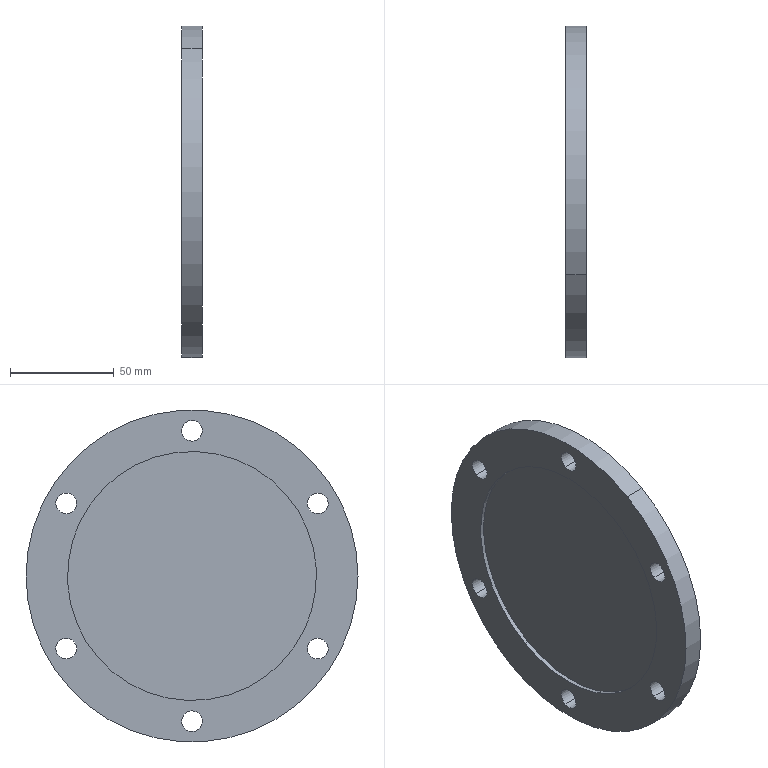Component | SolidWorks | GearboxEndCover-NoHole-2 | 1 solid | 19 faces | box 10 x 160 x 160 mm | volume 173730 mm3 | cylinder 16 | plane 3 | commonest cylinder face diameters 10 x12 120 x2 160 x2
build123d program:
from build123d import *

# Parameters (mm, degrees)
SKETCH1_3_R         = 80
SKETCH1_3_R_2       = 5
BOSS_EXTRUDE1_DEPTH = 8
BOSS_EXTRUDE2_START = -2
SKETCH1_3_2_R       = 80
SKETCH1_3_2_R_2     = 60
SKETCH1_3_2_R_3     = 5
BOSS_EXTRUDE2_DEPTH = 2


with BuildPart() as part:
    # Sketch1_3 → Boss-Extrude1 (new body)
    with BuildSketch(Plane(origin=(0, 0, 0), x_dir=(1, 0, 0), z_dir=(0, 1, 0))):
        with Locations(Location((0, 0, 0), (0, 0, 270))):
            Circle(SKETCH1_3_R)
        with Locations(Location((70, 0, 0), (0, 0, 270))):
            Circle(SKETCH1_3_R_2, mode=Mode.SUBTRACT)
        with Locations(Location((35, -60.622, 0), (0, 0, 270))):
            Circle(SKETCH1_3_R_2, mode=Mode.SUBTRACT)
        with Locations(Location((-35, -60.622, 0), (0, 0, 270))):
            Circle(SKETCH1_3_R_2, mode=Mode.SUBTRACT)
        with Locations(Location((-70, 0, 0), (0, 0, 270))):
            Circle(SKETCH1_3_R_2, mode=Mode.SUBTRACT)
        with Locations(Location((-35, 60.622, 0), (0, 0, 270))):
            Circle(SKETCH1_3_R_2, mode=Mode.SUBTRACT)
        with Locations(Location((35, 60.622, 0), (0, 0, 270))):
            Circle(SKETCH1_3_R_2, mode=Mode.SUBTRACT)
    extrude(amount=BOSS_EXTRUDE1_DEPTH)

    # Sketch1_3 2 → Boss-Extrude2 (add)
    with BuildSketch(Plane(origin=(0, 0, 0), x_dir=(1, 0, 0), z_dir=(0, 1, 0)).offset(BOSS_EXTRUDE2_START)):
        with Locations(Location((0, 0, 0), (0, 0, 270))):
            Circle(SKETCH1_3_2_R)
        with Locations(Location((0, 0, 0), (0, 0, 270))):
            Circle(SKETCH1_3_2_R_2, mode=Mode.SUBTRACT)
        with Locations(Location((70, 0, 0), (0, 0, 270))):
            Circle(SKETCH1_3_2_R_3, mode=Mode.SUBTRACT)
        with Locations(Location((35, -60.622, 0), (0, 0, 270))):
            Circle(SKETCH1_3_2_R_3, mode=Mode.SUBTRACT)
        with Locations(Location((-35, -60.622, 0), (0, 0, 270))):
            Circle(SKETCH1_3_2_R_3, mode=Mode.SUBTRACT)
        with Locations(Location((-70, 0, 0), (0, 0, 270))):
            Circle(SKETCH1_3_2_R_3, mode=Mode.SUBTRACT)
        with Locations(Location((-35, 60.622, 0), (0, 0, 270))):
            Circle(SKETCH1_3_2_R_3, mode=Mode.SUBTRACT)
        with Locations(Location((35, 60.622, 0), (0, 0, 270))):
            Circle(SKETCH1_3_2_R_3, mode=Mode.SUBTRACT)
    extrude(amount=BOSS_EXTRUDE2_DEPTH)


solid = part.part

# Placed as in the assembly
solid = solid.moved(Location((-178.429, -8.561, -165), (90, 0, -90)))
STEP:
#1=CARTESIAN_POINT('',(-7.104,0.844,-8.542));
#2=VERTEX_POINT('',#1);
#3=CARTESIAN_POINT('',(-7.104,-1.518,-4.45));
#4=VERTEX_POINT('',#3);
#5=CARTESIAN_POINT('',(-7.104,-0.3371,-6.496));
#6=DIRECTION('',(1.,0.,-0.));
#7=DIRECTION('',(0.,-0.5,0.866));
#8=AXIS2_PLACEMENT_3D('',#5,#6,#7);
#9=CIRCLE('',#8,2.362);
#10=EDGE_CURVE('',#2,#4,#9,.T.);
#11=ORIENTED_EDGE('',*,*,#10,.F.);
#12=CARTESIAN_POINT('',(-7.025,0.844,-8.542));
#13=VERTEX_POINT('',#12);
#14=CARTESIAN_POINT('',(-7.104,0.844,-8.542));
#15=DIRECTION('',(1.,0.,-0.));
#16=VECTOR('',#15,39.37);
#17=LINE('',#14,#16);
#18=EDGE_CURVE('',#2,#13,#17,.T.);
#19=ORIENTED_EDGE('',*,*,#18,.T.);
#20=CARTESIAN_POINT('',(-7.025,-1.518,-4.45));
#21=VERTEX_POINT('',#20);
#22=CARTESIAN_POINT('',(-7.025,-0.3371,-6.496));
#23=DIRECTION('',(1.,0.,-0.));
#24=DIRECTION('',(0.,-0.5,0.866));
#25=AXIS2_PLACEMENT_3D('',#22,#23,#24);
#26=CIRCLE('',#25,2.362);
#27=EDGE_CURVE('',#13,#21,#26,.T.);
#28=ORIENTED_EDGE('',*,*,#27,.T.);
#29=CARTESIAN_POINT('',(-7.104,-1.518,-4.45));
#30=DIRECTION('',(1.,0.,-0.));
#31=VECTOR('',#30,39.37);
#32=LINE('',#29,#31);
#33=EDGE_CURVE('',#4,#21,#32,.T.);
#34=ORIENTED_EDGE('',*,*,#33,.F.);
#35=EDGE_LOOP('',(#11,#19,#28,#34));
#36=FACE_OUTER_BOUND('',#35,.T.);
#37=CARTESIAN_POINT('',(-7.104,-0.3371,-6.496));
#38=DIRECTION('',(1.,0.,-0.));
#39=DIRECTION('',(0.,-0.5,0.866));
#40=AXIS2_PLACEMENT_3D('',#37,#38,#39);
#41=CYLINDRICAL_SURFACE('',#40,2.362);
#42=ADVANCED_FACE('',(#36),#41,.F.);
#43=CARTESIAN_POINT('',(-6.71,-1.912,-3.768));
#44=VERTEX_POINT('',#43);
#45=CARTESIAN_POINT('',(-6.71,1.238,-9.224));
#46=VERTEX_POINT('',#45);
#47=CARTESIAN_POINT('',(-6.71,-0.3371,-6.496));
#48=DIRECTION('',(1.,0.,-0.));
#49=DIRECTION('',(0.,-0.5,0.866));
#50=AXIS2_PLACEMENT_3D('',#47,#48,#49);
#51=CIRCLE('',#50,3.15);
#52=EDGE_CURVE('',#44,#46,#51,.T.);
#53=ORIENTED_EDGE('',*,*,#52,.F.);
#54=CARTESIAN_POINT('',(-7.104,-1.912,-3.768));
#55=VERTEX_POINT('',#54);
#56=CARTESIAN_POINT('',(-6.71,-1.912,-3.768));
#57=DIRECTION('',(-1.,-0.,0.));
#58=VECTOR('',#57,39.37);
#59=LINE('',#56,#58);
#60=EDGE_CURVE('',#44,#55,#59,.T.);
#61=ORIENTED_EDGE('',*,*,#60,.T.);
#62=CARTESIAN_POINT('',(-7.104,1.238,-9.224));
#63=VERTEX_POINT('',#62);
#64=CARTESIAN_POINT('',(-7.104,-0.3371,-6.496));
#65=DIRECTION('',(1.,0.,-0.));
#66=DIRECTION('',(0.,-0.5,0.866));
#67=AXIS2_PLACEMENT_3D('',#64,#65,#66);
#68=CIRCLE('',#67,3.15);
#69=EDGE_CURVE('',#55,#63,#68,.T.);
#70=ORIENTED_EDGE('',*,*,#69,.T.);
#71=CARTESIAN_POINT('',(-6.71,1.238,-9.224));
#72=DIRECTION('',(-1.,-0.,0.));
#73=VECTOR('',#72,39.37);
#74=LINE('',#71,#73);
#75=EDGE_CURVE('',#46,#63,#74,.T.);
#76=ORIENTED_EDGE('',*,*,#75,.F.);
#77=EDGE_LOOP('',(#53,#61,#70,#76));
#78=FACE_OUTER_BOUND('',#77,.T.);
#79=CARTESIAN_POINT('',(-6.71,-0.3371,-6.496));
#80=DIRECTION('',(-1.,-0.,0.));
#81=DIRECTION('',(0.,0.5,-0.866));
#82=AXIS2_PLACEMENT_3D('',#79,#80,#81);
#83=CYLINDRICAL_SURFACE('',#82,3.15);
#84=ADVANCED_FACE('',(#78),#83,.T.);
#85=CARTESIAN_POINT('',(-6.71,-2.625,-8.044));
#86=VERTEX_POINT('',#85);
#87=CARTESIAN_POINT('',(-6.71,-2.822,-7.704));
#88=VERTEX_POINT('',#87);
#89=CARTESIAN_POINT('',(-6.71,-2.724,-7.874));
#90=DIRECTION('',(1.,0.,-0.));
#91=DIRECTION('',(0.,-0.5,0.866));
#92=AXIS2_PLACEMENT_3D('',#89,#90,#91);
#93=CIRCLE('',#92,0.1969);
#94=EDGE_CURVE('',#86,#88,#93,.T.);
#95=ORIENTED_EDGE('',*,*,#94,.T.);
#96=CARTESIAN_POINT('',(-7.104,-2.822,-7.704));
#97=VERTEX_POINT('',#96);
#98=CARTESIAN_POINT('',(-6.71,-2.822,-7.704));
#99=DIRECTION('',(-1.,-0.,0.));
#100=VECTOR('',#99,39.37);
#101=LINE('',#98,#100);
#102=EDGE_CURVE('',#88,#97,#101,.T.);
#103=ORIENTED_EDGE('',*,*,#102,.T.);
#104=CARTESIAN_POINT('',(-7.104,-2.625,-8.044));
#105=VERTEX_POINT('',#104);
#106=CARTESIAN_POINT('',(-7.104,-2.724,-7.874));
#107=DIRECTION('',(1.,0.,-0.));
#108=DIRECTION('',(0.,-0.5,0.866));
#109=AXIS2_PLACEMENT_3D('',#106,#107,#108);
#110=CIRCLE('',#109,0.1969);
#111=EDGE_CURVE('',#105,#97,#110,.T.);
#112=ORIENTED_EDGE('',*,*,#111,.F.);
#113=CARTESIAN_POINT('',(-6.71,-2.625,-8.044));
#114=DIRECTION('',(-1.,-0.,0.));
#115=VECTOR('',#114,39.37);
#116=LINE('',#113,#115);
#117=EDGE_CURVE('',#86,#105,#116,.T.);
#118=ORIENTED_EDGE('',*,*,#117,.F.);
#119=EDGE_LOOP('',(#95,#103,#112,#118));
#120=FACE_OUTER_BOUND('',#119,.T.);
#121=CARTESIAN_POINT('',(-6.71,-2.724,-7.874));
#122=DIRECTION('',(-1.,-0.,0.));
#123=DIRECTION('',(0.,0.5,-0.866));
#124=AXIS2_PLACEMENT_3D('',#121,#122,#123);
#125=CYLINDRICAL_SURFACE('',#124,0.1969);
#126=ADVANCED_FACE('',(#120),#125,.F.);
#127=CARTESIAN_POINT('',(-6.71,-0.2386,-9.422));
#128=VERTEX_POINT('',#127);
#129=CARTESIAN_POINT('',(-6.71,-0.4355,-9.081));
#130=VERTEX_POINT('',#129);
#131=CARTESIAN_POINT('',(-6.71,-0.3371,-9.252));
#132=DIRECTION('',(1.,0.,-0.));
#133=DIRECTION('',(0.,-0.5,0.866));
#134=AXIS2_PLACEMENT_3D('',#131,#132,#133);
#135=CIRCLE('',#134,0.1969);
#136=EDGE_CURVE('',#128,#130,#135,.T.);
#137=ORIENTED_EDGE('',*,*,#136,.T.);
#138=CARTESIAN_POINT('',(-7.104,-0.4355,-9.081));
#139=VERTEX_POINT('',#138);
#140=CARTESIAN_POINT('',(-6.71,-0.4355,-9.081));
#141=DIRECTION('',(-1.,-0.,0.));
#142=VECTOR('',#141,39.37);
#143=LINE('',#140,#142);
#144=EDGE_CURVE('',#130,#139,#143,.T.);
#145=ORIENTED_EDGE('',*,*,#144,.T.);
#146=CARTESIAN_POINT('',(-7.104,-0.2386,-9.422));
#147=VERTEX_POINT('',#146);
#148=CARTESIAN_POINT('',(-7.104,-0.3371,-9.252));
#149=DIRECTION('',(1.,0.,-0.));
#150=DIRECTION('',(0.,-0.5,0.866));
#151=AXIS2_PLACEMENT_3D('',#148,#149,#150);
#152=CIRCLE('',#151,0.1969);
#153=EDGE_CURVE('',#147,#139,#152,.T.);
#154=ORIENTED_EDGE('',*,*,#153,.F.);
#155=CARTESIAN_POINT('',(-6.71,-0.2386,-9.422));
#156=DIRECTION('',(-1.,-0.,0.));
#157=VECTOR('',#156,39.37);
#158=LINE('',#155,#157);
#159=EDGE_CURVE('',#128,#147,#158,.T.);
#160=ORIENTED_EDGE('',*,*,#159,.F.);
#161=EDGE_LOOP('',(#137,#145,#154,#160));
#162=FACE_OUTER_BOUND('',#161,.T.);
#163=CARTESIAN_POINT('',(-6.71,-0.3371,-9.252));
#164=DIRECTION('',(-1.,-0.,0.));
#165=DIRECTION('',(0.,0.5,-0.866));
#166=AXIS2_PLACEMENT_3D('',#163,#164,#165);
#167=CYLINDRICAL_SURFACE('',#166,0.1969);
#168=ADVANCED_FACE('',(#162),#167,.F.);
#169=CARTESIAN_POINT('',(-6.71,2.148,-8.044));
#170=VERTEX_POINT('',#169);
#171=CARTESIAN_POINT('',(-6.71,1.951,-7.704));
#172=VERTEX_POINT('',#171);
#173=CARTESIAN_POINT('',(-6.71,2.05,-7.874));
#174=DIRECTION('',(1.,0.,-0.));
#175=DIRECTION('',(0.,-0.5,0.866));
#176=AXIS2_PLACEMENT_3D('',#173,#174,#175);
#177=CIRCLE('',#176,0.1969);
#178=EDGE_CURVE('',#170,#172,#177,.T.);
#179=ORIENTED_EDGE('',*,*,#178,.T.);
#180=CARTESIAN_POINT('',(-7.104,1.951,-7.704));
#181=VERTEX_POINT('',#180);
#182=CARTESIAN_POINT('',(-6.71,1.951,-7.704));
#183=DIRECTION('',(-1.,-0.,0.));
#184=VECTOR('',#183,39.37);
#185=LINE('',#182,#184);
#186=EDGE_CURVE('',#172,#181,#185,.T.);
#187=ORIENTED_EDGE('',*,*,#186,.T.);
#188=CARTESIAN_POINT('',(-7.104,2.148,-8.044));
#189=VERTEX_POINT('',#188);
#190=CARTESIAN_POINT('',(-7.104,2.05,-7.874));
#191=DIRECTION('',(1.,0.,-0.));
#192=DIRECTION('',(0.,-0.5,0.866));
#193=AXIS2_PLACEMENT_3D('',#190,#191,#192);
#194=CIRCLE('',#193,0.1969);
#195=EDGE_CURVE('',#189,#181,#194,.T.);
#196=ORIENTED_EDGE('',*,*,#195,.F.);
#197=CARTESIAN_POINT('',(-6.71,2.148,-8.044));
#198=DIRECTION('',(-1.,-0.,0.));
#199=VECTOR('',#198,39.37);
#200=LINE('',#197,#199);
#201=EDGE_CURVE('',#170,#189,#200,.T.);
#202=ORIENTED_EDGE('',*,*,#201,.F.);
#203=EDGE_LOOP('',(#179,#187,#196,#202));
#204=FACE_OUTER_BOUND('',#203,.T.);
#205=CARTESIAN_POINT('',(-6.71,2.05,-7.874));
#206=DIRECTION('',(-1.,-0.,0.));
#207=DIRECTION('',(0.,0.5,-0.866));
#208=AXIS2_PLACEMENT_3D('',#205,#206,#207);
#209=CYLINDRICAL_SURFACE('',#208,0.1969);
#210=ADVANCED_FACE('',(#204),#209,.F.);
#211=CARTESIAN_POINT('',(-6.71,2.148,-5.289));
#212=VERTEX_POINT('',#211);
#213=CARTESIAN_POINT('',(-6.71,1.951,-4.948));
#214=VERTEX_POINT('',#213);
#215=CARTESIAN_POINT('',(-6.71,2.05,-5.118));
#216=DIRECTION('',(1.,0.,-0.));
#217=DIRECTION('',(0.,-0.5,0.866));
#218=AXIS2_PLACEMENT_3D('',#215,#216,#217);
#219=CIRCLE('',#218,0.1969);
#220=EDGE_CURVE('',#212,#214,#219,.T.);
#221=ORIENTED_EDGE('',*,*,#220,.T.);
#222=CARTESIAN_POINT('',(-7.104,1.951,-4.948));
#223=VERTEX_POINT('',#222);
#224=CARTESIAN_POINT('',(-6.71,1.951,-4.948));
#225=DIRECTION('',(-1.,-0.,0.));
#226=VECTOR('',#225,39.37);
#227=LINE('',#224,#226);
#228=EDGE_CURVE('',#214,#223,#227,.T.);
#229=ORIENTED_EDGE('',*,*,#228,.T.);
#230=CARTESIAN_POINT('',(-7.104,2.148,-5.289));
#231=VERTEX_POINT('',#230);
#232=CARTESIAN_POINT('',(-7.104,2.05,-5.118));
#233=DIRECTION('',(1.,0.,-0.));
#234=DIRECTION('',(0.,-0.5,0.866));
#235=AXIS2_PLACEMENT_3D('',#232,#233,#234);
#236=CIRCLE('',#235,0.1969);
#237=EDGE_CURVE('',#231,#223,#236,.T.);
#238=ORIENTED_EDGE('',*,*,#237,.F.);
#239=CARTESIAN_POINT('',(-6.71,2.148,-5.289));
#240=DIRECTION('',(-1.,-0.,0.));
#241=VECTOR('',#240,39.37);
#242=LINE('',#239,#241);
#243=EDGE_CURVE('',#212,#231,#242,.T.);
#244=ORIENTED_EDGE('',*,*,#243,.F.);
#245=EDGE_LOOP('',(#221,#229,#238,#244));
#246=FACE_OUTER_BOUND('',#245,.T.);
#247=CARTESIAN_POINT('',(-6.71,2.05,-5.118));
#248=DIRECTION('',(-1.,-0.,0.));
#249=DIRECTION('',(0.,0.5,-0.866));
#250=AXIS2_PLACEMENT_3D('',#247,#248,#249);
#251=CYLINDRICAL_SURFACE('',#250,0.1969);
#252=ADVANCED_FACE('',(#246),#251,.F.);
#253=CARTESIAN_POINT('',(-6.71,-0.2386,-3.911));
#254=VERTEX_POINT('',#253);
#255=CARTESIAN_POINT('',(-6.71,-0.4355,-3.57));
#256=VERTEX_POINT('',#255);
#257=CARTESIAN_POINT('',(-6.71,-0.3371,-3.74));
#258=DIRECTION('',(1.,0.,-0.));
#259=DIRECTION('',(0.,-0.5,0.866));
#260=AXIS2_PLACEMENT_3D('',#257,#258,#259);
#261=CIRCLE('',#260,0.1969);
#262=EDGE_CURVE('',#254,#256,#261,.T.);
#263=ORIENTED_EDGE('',*,*,#262,.T.);
#264=CARTESIAN_POINT('',(-7.104,-0.4355,-3.57));
#265=VERTEX_POINT('',#264);
#266=CARTESIAN_POINT('',(-6.71,-0.4355,-3.57));
#267=DIRECTION('',(-1.,-0.,0.));
#268=VECTOR('',#267,39.37);
#269=LINE('',#266,#268);
#270=EDGE_CURVE('',#256,#265,#269,.T.);
#271=ORIENTED_EDGE('',*,*,#270,.T.);
#272=CARTESIAN_POINT('',(-7.104,-0.2386,-3.911));
#273=VERTEX_POINT('',#272);
#274=CARTESIAN_POINT('',(-7.104,-0.3371,-3.74));
#275=DIRECTION('',(1.,0.,-0.));
#276=DIRECTION('',(0.,-0.5,0.866));
#277=AXIS2_PLACEMENT_3D('',#274,#275,#276);
#278=CIRCLE('',#277,0.1969);
#279=EDGE_CURVE('',#273,#265,#278,.T.);
#280=ORIENTED_EDGE('',*,*,#279,.F.);
#281=CARTESIAN_POINT('',(-6.71,-0.2386,-3.911));
#282=DIRECTION('',(-1.,-0.,0.));
#283=VECTOR('',#282,39.37);
#284=LINE('',#281,#283);
#285=EDGE_CURVE('',#254,#273,#284,.T.);
#286=ORIENTED_EDGE('',*,*,#285,.F.);
#287=EDGE_LOOP('',(#263,#271,#280,#286));
#288=FACE_OUTER_BOUND('',#287,.T.);
#289=CARTESIAN_POINT('',(-6.71,-0.3371,-3.74));
#290=DIRECTION('',(-1.,-0.,0.));
#291=DIRECTION('',(0.,0.5,-0.866));
#292=AXIS2_PLACEMENT_3D('',#289,#290,#291);
#293=CYLINDRICAL_SURFACE('',#292,0.1969);
#294=ADVANCED_FACE('',(#288),#293,.F.);
#295=CARTESIAN_POINT('',(-6.71,-2.625,-5.289));
#296=VERTEX_POINT('',#295);
#297=CARTESIAN_POINT('',(-6.71,-2.822,-4.948));
#298=VERTEX_POINT('',#297);
#299=CARTESIAN_POINT('',(-6.71,-2.724,-5.118));
#300=DIRECTION('',(1.,0.,-0.));
#301=DIRECTION('',(0.,-0.5,0.866));
#302=AXIS2_PLACEMENT_3D('',#299,#300,#301);
#303=CIRCLE('',#302,0.1969);
#304=EDGE_CURVE('',#296,#298,#303,.T.);
#305=ORIENTED_EDGE('',*,*,#304,.T.);
#306=CARTESIAN_POINT('',(-7.104,-2.822,-4.948));
#307=VERTEX_POINT('',#306);
#308=CARTESIAN_POINT('',(-6.71,-2.822,-4.948));
#309=DIRECTION('',(-1.,-0.,0.));
#310=VECTOR('',#309,39.37);
#311=LINE('',#308,#310);
#312=EDGE_CURVE('',#298,#307,#311,.T.);
#313=ORIENTED_EDGE('',*,*,#312,.T.);
#314=CARTESIAN_POINT('',(-7.104,-2.625,-5.289));
#315=VERTEX_POINT('',#314);
#316=CARTESIAN_POINT('',(-7.104,-2.724,-5.118));
#317=DIRECTION('',(1.,0.,-0.));
#318=DIRECTION('',(0.,-0.5,0.866));
#319=AXIS2_PLACEMENT_3D('',#316,#317,#318);
#320=CIRCLE('',#319,0.1969);
#321=EDGE_CURVE('',#315,#307,#320,.T.);
#322=ORIENTED_EDGE('',*,*,#321,.F.);
#323=CARTESIAN_POINT('',(-6.71,-2.625,-5.289));
#324=DIRECTION('',(-1.,-0.,0.));
#325=VECTOR('',#324,39.37);
#326=LINE('',#323,#325);
#327=EDGE_CURVE('',#296,#315,#326,.T.);
#328=ORIENTED_EDGE('',*,*,#327,.F.);
#329=EDGE_LOOP('',(#305,#313,#322,#328));
#330=FACE_OUTER_BOUND('',#329,.T.);
#331=CARTESIAN_POINT('',(-6.71,-2.724,-5.118));
#332=DIRECTION('',(-1.,-0.,0.));
#333=DIRECTION('',(0.,0.5,-0.866));
#334=AXIS2_PLACEMENT_3D('',#331,#332,#333);
#335=CYLINDRICAL_SURFACE('',#334,0.1969);
#336=ADVANCED_FACE('',(#330),#335,.F.);
#337=ORIENTED_EDGE('',*,*,#312,.F.);
#338=CARTESIAN_POINT('',(-6.71,-2.724,-5.118));
#339=DIRECTION('',(1.,0.,-0.));
#340=DIRECTION('',(0.,-0.5,0.866));
#341=AXIS2_PLACEMENT_3D('',#338,#339,#340);
#342=CIRCLE('',#341,0.1969);
#343=EDGE_CURVE('',#298,#296,#342,.T.);
#344=ORIENTED_EDGE('',*,*,#343,.T.);
#345=ORIENTED_EDGE('',*,*,#327,.T.);
#346=CARTESIAN_POINT('',(-7.104,-2.724,-5.118));
#347=DIRECTION('',(1.,0.,-0.));
#348=DIRECTION('',(0.,-0.5,0.866));
#349=AXIS2_PLACEMENT_3D('',#346,#347,#348);
#350=CIRCLE('',#349,0.1969);
#351=EDGE_CURVE('',#307,#315,#350,.T.);
#352=ORIENTED_EDGE('',*,*,#351,.F.);
#353=EDGE_LOOP('',(#337,#344,#345,#352));
#354=FACE_OUTER_BOUND('',#353,.T.);
#355=CARTESIAN_POINT('',(-6.71,-2.724,-5.118));
#356=DIRECTION('',(-1.,-0.,0.));
#357=DIRECTION('',(0.,0.5,-0.866));
#358=AXIS2_PLACEMENT_3D('',#355,#356,#357);
#359=CYLINDRICAL_SURFACE('',#358,0.1969);
#360=ADVANCED_FACE('',(#354),#359,.F.);
#361=ORIENTED_EDGE('',*,*,#270,.F.);
#362=CARTESIAN_POINT('',(-6.71,-0.3371,-3.74));
#363=DIRECTION('',(1.,0.,-0.));
#364=DIRECTION('',(0.,-0.5,0.866));
#365=AXIS2_PLACEMENT_3D('',#362,#363,#364);
#366=CIRCLE('',#365,0.1969);
#367=EDGE_CURVE('',#256,#254,#366,.T.);
#368=ORIENTED_EDGE('',*,*,#367,.T.);
#369=ORIENTED_EDGE('',*,*,#285,.T.);
#370=CARTESIAN_POINT('',(-7.104,-0.3371,-3.74));
#371=DIRECTION('',(1.,0.,-0.));
#372=DIRECTION('',(0.,-0.5,0.866));
#373=AXIS2_PLACEMENT_3D('',#370,#371,#372);
#374=CIRCLE('',#373,0.1969);
#375=EDGE_CURVE('',#265,#273,#374,.T.);
#376=ORIENTED_EDGE('',*,*,#375,.F.);
#377=EDGE_LOOP('',(#361,#368,#369,#376));
#378=FACE_OUTER_BOUND('',#377,.T.);
#379=CARTESIAN_POINT('',(-6.71,-0.3371,-3.74));
#380=DIRECTION('',(-1.,-0.,0.));
#381=DIRECTION('',(0.,0.5,-0.866));
#382=AXIS2_PLACEMENT_3D('',#379,#380,#381);
#383=CYLINDRICAL_SURFACE('',#382,0.1969);
#384=ADVANCED_FACE('',(#378),#383,.F.);
#385=ORIENTED_EDGE('',*,*,#228,.F.);
#386=CARTESIAN_POINT('',(-6.71,2.05,-5.118));
#387=DIRECTION('',(1.,0.,-0.));
#388=DIRECTION('',(0.,-0.5,0.866));
#389=AXIS2_PLACEMENT_3D('',#386,#387,#388);
#390=CIRCLE('',#389,0.1969);
#391=EDGE_CURVE('',#214,#212,#390,.T.);
#392=ORIENTED_EDGE('',*,*,#391,.T.);
#393=ORIENTED_EDGE('',*,*,#243,.T.);
#394=CARTESIAN_POINT('',(-7.104,2.05,-5.118));
#395=DIRECTION('',(1.,0.,-0.));
#396=DIRECTION('',(0.,-0.5,0.866));
#397=AXIS2_PLACEMENT_3D('',#394,#395,#396);
#398=CIRCLE('',#397,0.1969);
#399=EDGE_CURVE('',#223,#231,#398,.T.);
#400=ORIENTED_EDGE('',*,*,#399,.F.);
#401=EDGE_LOOP('',(#385,#392,#393,#400));
#402=FACE_OUTER_BOUND('',#401,.T.);
#403=CARTESIAN_POINT('',(-6.71,2.05,-5.118));
#404=DIRECTION('',(-1.,-0.,0.));
#405=DIRECTION('',(0.,0.5,-0.866));
#406=AXIS2_PLACEMENT_3D('',#403,#404,#405);
#407=CYLINDRICAL_SURFACE('',#406,0.1969);
#408=ADVANCED_FACE('',(#402),#407,.F.);
#409=ORIENTED_EDGE('',*,*,#186,.F.);
#410=CARTESIAN_POINT('',(-6.71,2.05,-7.874));
#411=DIRECTION('',(1.,0.,-0.));
#412=DIRECTION('',(0.,-0.5,0.866));
#413=AXIS2_PLACEMENT_3D('',#410,#411,#412);
#414=CIRCLE('',#413,0.1969);
#415=EDGE_CURVE('',#172,#170,#414,.T.);
#416=ORIENTED_EDGE('',*,*,#415,.T.);
#417=ORIENTED_EDGE('',*,*,#201,.T.);
#418=CARTESIAN_POINT('',(-7.104,2.05,-7.874));
#419=DIRECTION('',(1.,0.,-0.));
#420=DIRECTION('',(0.,-0.5,0.866));
#421=AXIS2_PLACEMENT_3D('',#418,#419,#420);
#422=CIRCLE('',#421,0.1969);
#423=EDGE_CURVE('',#181,#189,#422,.T.);
#424=ORIENTED_EDGE('',*,*,#423,.F.);
#425=EDGE_LOOP('',(#409,#416,#417,#424));
#426=FACE_OUTER_BOUND('',#425,.T.);
#427=CARTESIAN_POINT('',(-6.71,2.05,-7.874));
#428=DIRECTION('',(-1.,-0.,0.));
#429=DIRECTION('',(0.,0.5,-0.866));
#430=AXIS2_PLACEMENT_3D('',#427,#428,#429);
#431=CYLINDRICAL_SURFACE('',#430,0.1969);
#432=ADVANCED_FACE('',(#426),#431,.F.);
#433=ORIENTED_EDGE('',*,*,#144,.F.);
#434=CARTESIAN_POINT('',(-6.71,-0.3371,-9.252));
#435=DIRECTION('',(1.,0.,-0.));
#436=DIRECTION('',(0.,-0.5,0.866));
#437=AXIS2_PLACEMENT_3D('',#434,#435,#436);
#438=CIRCLE('',#437,0.1969);
#439=EDGE_CURVE('',#130,#128,#438,.T.);
#440=ORIENTED_EDGE('',*,*,#439,.T.);
#441=ORIENTED_EDGE('',*,*,#159,.T.);
#442=CARTESIAN_POINT('',(-7.104,-0.3371,-9.252));
#443=DIRECTION('',(1.,0.,-0.));
#444=DIRECTION('',(0.,-0.5,0.866));
#445=AXIS2_PLACEMENT_3D('',#442,#443,#444);
#446=CIRCLE('',#445,0.1969);
#447=EDGE_CURVE('',#139,#147,#446,.T.);
#448=ORIENTED_EDGE('',*,*,#447,.F.);
#449=EDGE_LOOP('',(#433,#440,#441,#448));
#450=FACE_OUTER_BOUND('',#449,.T.);
#451=CARTESIAN_POINT('',(-6.71,-0.3371,-9.252));
#452=DIRECTION('',(-1.,-0.,0.));
#453=DIRECTION('',(0.,0.5,-0.866));
#454=AXIS2_PLACEMENT_3D('',#451,#452,#453);
#455=CYLINDRICAL_SURFACE('',#454,0.1969);
#456=ADVANCED_FACE('',(#450),#455,.F.);
#457=ORIENTED_EDGE('',*,*,#102,.F.);
#458=CARTESIAN_POINT('',(-6.71,-2.724,-7.874));
#459=DIRECTION('',(1.,0.,-0.));
#460=DIRECTION('',(0.,-0.5,0.866));
#461=AXIS2_PLACEMENT_3D('',#458,#459,#460);
#462=CIRCLE('',#461,0.1969);
#463=EDGE_CURVE('',#88,#86,#462,.T.);
#464=ORIENTED_EDGE('',*,*,#463,.T.);
#465=ORIENTED_EDGE('',*,*,#117,.T.);
#466=CARTESIAN_POINT('',(-7.104,-2.724,-7.874));
#467=DIRECTION('',(1.,0.,-0.));
#468=DIRECTION('',(0.,-0.5,0.866));
#469=AXIS2_PLACEMENT_3D('',#466,#467,#468);
#470=CIRCLE('',#469,0.1969);
#471=EDGE_CURVE('',#97,#105,#470,.T.);
#472=ORIENTED_EDGE('',*,*,#471,.F.);
#473=EDGE_LOOP('',(#457,#464,#465,#472));
#474=FACE_OUTER_BOUND('',#473,.T.);
#475=CARTESIAN_POINT('',(-6.71,-2.724,-7.874));
#476=DIRECTION('',(-1.,-0.,0.));
#477=DIRECTION('',(0.,0.5,-0.866));
#478=AXIS2_PLACEMENT_3D('',#475,#476,#477);
#479=CYLINDRICAL_SURFACE('',#478,0.1969);
#480=ADVANCED_FACE('',(#474),#479,.F.);
#481=ORIENTED_EDGE('',*,*,#60,.F.);
#482=CARTESIAN_POINT('',(-6.71,-0.3371,-6.496));
#483=DIRECTION('',(1.,0.,-0.));
#484=DIRECTION('',(0.,-0.5,0.866));
#485=AXIS2_PLACEMENT_3D('',#482,#483,#484);
#486=CIRCLE('',#485,3.15);
#487=EDGE_CURVE('',#46,#44,#486,.T.);
#488=ORIENTED_EDGE('',*,*,#487,.F.);
#489=ORIENTED_EDGE('',*,*,#75,.T.);
#490=CARTESIAN_POINT('',(-7.104,-0.3371,-6.496));
#491=DIRECTION('',(1.,0.,-0.));
#492=DIRECTION('',(0.,-0.5,0.866));
#493=AXIS2_PLACEMENT_3D('',#490,#491,#492);
#494=CIRCLE('',#493,3.15);
#495=EDGE_CURVE('',#63,#55,#494,.T.);
#496=ORIENTED_EDGE('',*,*,#495,.T.);
#497=EDGE_LOOP('',(#481,#488,#489,#496));
#498=FACE_OUTER_BOUND('',#497,.T.);
#499=CARTESIAN_POINT('',(-6.71,-0.3371,-6.496));
#500=DIRECTION('',(-1.,-0.,0.));
#501=DIRECTION('',(0.,0.5,-0.866));
#502=AXIS2_PLACEMENT_3D('',#499,#500,#501);
#503=CYLINDRICAL_SURFACE('',#502,3.15);
#504=ADVANCED_FACE('',(#498),#503,.T.);
#505=ORIENTED_EDGE('',*,*,#94,.F.);
#506=ORIENTED_EDGE('',*,*,#463,.F.);
#507=EDGE_LOOP('',(#505,#506));
#508=FACE_BOUND('',#507,.T.);
#509=ORIENTED_EDGE('',*,*,#136,.F.);
#510=ORIENTED_EDGE('',*,*,#439,.F.);
#511=EDGE_LOOP('',(#509,#510));
#512=FACE_BOUND('',#511,.T.);
#513=ORIENTED_EDGE('',*,*,#178,.F.);
#514=ORIENTED_EDGE('',*,*,#415,.F.);
#515=EDGE_LOOP('',(#513,#514));
#516=FACE_BOUND('',#515,.T.);
#517=ORIENTED_EDGE('',*,*,#220,.F.);
#518=ORIENTED_EDGE('',*,*,#391,.F.);
#519=EDGE_LOOP('',(#517,#518));
#520=FACE_BOUND('',#519,.T.);
#521=ORIENTED_EDGE('',*,*,#262,.F.);
#522=ORIENTED_EDGE('',*,*,#367,.F.);
#523=EDGE_LOOP('',(#521,#522));
#524=FACE_BOUND('',#523,.T.);
#525=ORIENTED_EDGE('',*,*,#304,.F.);
#526=ORIENTED_EDGE('',*,*,#343,.F.);
#527=EDGE_LOOP('',(#525,#526));
#528=FACE_BOUND('',#527,.T.);
#529=ORIENTED_EDGE('',*,*,#487,.T.);
#530=ORIENTED_EDGE('',*,*,#52,.T.);
#531=EDGE_LOOP('',(#529,#530));
#532=FACE_OUTER_BOUND('',#531,.T.);
#533=CARTESIAN_POINT('',(-6.71,5.669,-3.029));
#534=DIRECTION('',(1.,0.,-0.));
#535=DIRECTION('',(0.,-0.5,0.866));
#536=AXIS2_PLACEMENT_3D('',#533,#534,#535);
#537=PLANE('',#536);
#538=ADVANCED_FACE('',(#508,#512,#516,#520,#524,#528,#532),#537,.T.);
#539=ORIENTED_EDGE('',*,*,#18,.F.);
#540=CARTESIAN_POINT('',(-7.104,-0.3371,-6.496));
#541=DIRECTION('',(1.,0.,-0.));
#542=DIRECTION('',(0.,-0.5,0.866));
#543=AXIS2_PLACEMENT_3D('',#540,#541,#542);
#544=CIRCLE('',#543,2.362);
#545=EDGE_CURVE('',#4,#2,#544,.T.);
#546=ORIENTED_EDGE('',*,*,#545,.F.);
#547=ORIENTED_EDGE('',*,*,#33,.T.);
#548=CARTESIAN_POINT('',(-7.025,-0.3371,-6.496));
#549=DIRECTION('',(1.,0.,-0.));
#550=DIRECTION('',(0.,-0.5,0.866));
#551=AXIS2_PLACEMENT_3D('',#548,#549,#550);
#552=CIRCLE('',#551,2.362);
#553=EDGE_CURVE('',#21,#13,#552,.T.);
#554=ORIENTED_EDGE('',*,*,#553,.T.);
#555=EDGE_LOOP('',(#539,#546,#547,#554));
#556=FACE_OUTER_BOUND('',#555,.T.);
#557=CARTESIAN_POINT('',(-7.104,-0.3371,-6.496));
#558=DIRECTION('',(1.,0.,-0.));
#559=DIRECTION('',(0.,-0.5,0.866));
#560=AXIS2_PLACEMENT_3D('',#557,#558,#559);
#561=CYLINDRICAL_SURFACE('',#560,2.362);
#562=ADVANCED_FACE('',(#556),#561,.F.);
#563=ORIENTED_EDGE('',*,*,#111,.T.);
#564=ORIENTED_EDGE('',*,*,#471,.T.);
#565=EDGE_LOOP('',(#563,#564));
#566=FACE_BOUND('',#565,.T.);
#567=ORIENTED_EDGE('',*,*,#153,.T.);
#568=ORIENTED_EDGE('',*,*,#447,.T.);
#569=EDGE_LOOP('',(#567,#568));
#570=FACE_BOUND('',#569,.T.);
#571=ORIENTED_EDGE('',*,*,#195,.T.);
#572=ORIENTED_EDGE('',*,*,#423,.T.);
#573=EDGE_LOOP('',(#571,#572));
#574=FACE_BOUND('',#573,.T.);
#575=ORIENTED_EDGE('',*,*,#237,.T.);
#576=ORIENTED_EDGE('',*,*,#399,.T.);
#577=EDGE_LOOP('',(#575,#576));
#578=FACE_BOUND('',#577,.T.);
#579=ORIENTED_EDGE('',*,*,#279,.T.);
#580=ORIENTED_EDGE('',*,*,#375,.T.);
#581=EDGE_LOOP('',(#579,#580));
#582=FACE_BOUND('',#581,.T.);
#583=ORIENTED_EDGE('',*,*,#321,.T.);
#584=ORIENTED_EDGE('',*,*,#351,.T.);
#585=EDGE_LOOP('',(#583,#584));
#586=FACE_BOUND('',#585,.T.);
#587=ORIENTED_EDGE('',*,*,#545,.T.);
#588=ORIENTED_EDGE('',*,*,#10,.T.);
#589=EDGE_LOOP('',(#587,#588));
#590=FACE_BOUND('',#589,.T.);
#591=ORIENTED_EDGE('',*,*,#495,.F.);
#592=ORIENTED_EDGE('',*,*,#69,.F.);
#593=EDGE_LOOP('',(#591,#592));
#594=FACE_OUTER_BOUND('',#593,.T.);
#595=CARTESIAN_POINT('',(-7.104,5.669,-3.029));
#596=DIRECTION('',(1.,0.,-0.));
#597=DIRECTION('',(0.,-0.5,0.866));
#598=AXIS2_PLACEMENT_3D('',#595,#596,#597);
#599=PLANE('',#598);
#600=ADVANCED_FACE('',(#566,#570,#574,#578,#582,#586,#590,#594),#599,.F.);
#601=ORIENTED_EDGE('',*,*,#553,.F.);
#602=ORIENTED_EDGE('',*,*,#27,.F.);
#603=EDGE_LOOP('',(#601,#602));
#604=FACE_OUTER_BOUND('',#603,.T.);
#605=CARTESIAN_POINT('',(-7.025,5.669,-3.029));
#606=DIRECTION('',(1.,0.,-0.));
#607=DIRECTION('',(0.,-0.5,0.866));
#608=AXIS2_PLACEMENT_3D('',#605,#606,#607);
#609=PLANE('',#608);
#610=ADVANCED_FACE('',(#604),#609,.F.);
#611=CLOSED_SHELL('',(#42,#84,#126,#168,#210,#252,#294,#336,#360,#384,#408,#432,#456,#480,#504,#538,#562,#600,#610));
#612=MANIFOLD_SOLID_BREP('',#611);
#613=CARTESIAN_POINT('',(0.,0.,0.));
#614=DIRECTION('',(0.,0.,1.));
#615=DIRECTION('',(1.,0.,0.));
#616=AXIS2_PLACEMENT_3D('',#613,#614,#615);
#617=(LENGTH_UNIT()NAMED_UNIT(*)SI_UNIT($,.METRE.));
#618=LENGTH_MEASURE_WITH_UNIT(LENGTH_MEASURE(0.0254),#617);
#619=DIMENSIONAL_EXPONENTS(1.,0.,0.,0.,0.,0.,0.);
#620=(CONVERSION_BASED_UNIT('',#618)LENGTH_UNIT()NAMED_UNIT(#619));
#621=UNCERTAINTY_MEASURE_WITH_UNIT(LENGTH_MEASURE(0.00001),#620,'','');
#622=(NAMED_UNIT(*)PLANE_ANGLE_UNIT()SI_UNIT($,.RADIAN.));
#623=(NAMED_UNIT(*)SI_UNIT($,.STERADIAN.)SOLID_ANGLE_UNIT());
#624=(GEOMETRIC_REPRESENTATION_CONTEXT(3)GLOBAL_UNCERTAINTY_ASSIGNED_CONTEXT((#621))GLOBAL_UNIT_ASSIGNED_CONTEXT((#620,#622,#623))REPRESENTATION_CONTEXT('',''));
#625=ADVANCED_BREP_SHAPE_REPRESENTATION('',(#612,#616),#624);
#626=COLOUR_RGB('',0.7922,0.8196,0.9333);
#627=FILL_AREA_STYLE_COLOUR('',#626);
#628=FILL_AREA_STYLE('',(#627));
#629=SURFACE_STYLE_FILL_AREA(#628);
#630=SURFACE_SIDE_STYLE('',(#629));
#631=SURFACE_STYLE_USAGE(.BOTH.,#630);
#632=PRESENTATION_STYLE_ASSIGNMENT((#631));
#633=STYLED_ITEM('',(#632),#612);
#634=PRESENTATION_LAYER_ASSIGNMENT('','',(#633));
#635=(LENGTH_UNIT()NAMED_UNIT(*)SI_UNIT($,.METRE.));
#636=LENGTH_MEASURE_WITH_UNIT(LENGTH_MEASURE(0.0254),#635);
#637=DIMENSIONAL_EXPONENTS(1.,0.,0.,0.,0.,0.,0.);
#638=(CONVERSION_BASED_UNIT('',#636)LENGTH_UNIT()NAMED_UNIT(#637));
#639=UNCERTAINTY_MEASURE_WITH_UNIT(LENGTH_MEASURE(0.00001),#638,'','');
#640=(NAMED_UNIT(*)PLANE_ANGLE_UNIT()SI_UNIT($,.RADIAN.));
#641=(NAMED_UNIT(*)SI_UNIT($,.STERADIAN.)SOLID_ANGLE_UNIT());
#642=(GEOMETRIC_REPRESENTATION_CONTEXT(3)GLOBAL_UNCERTAINTY_ASSIGNED_CONTEXT((#639))GLOBAL_UNIT_ASSIGNED_CONTEXT((#638,#640,#641))REPRESENTATION_CONTEXT('',''));
#643=MECHANICAL_DESIGN_GEOMETRIC_PRESENTATION_REPRESENTATION('',(#633),#642);